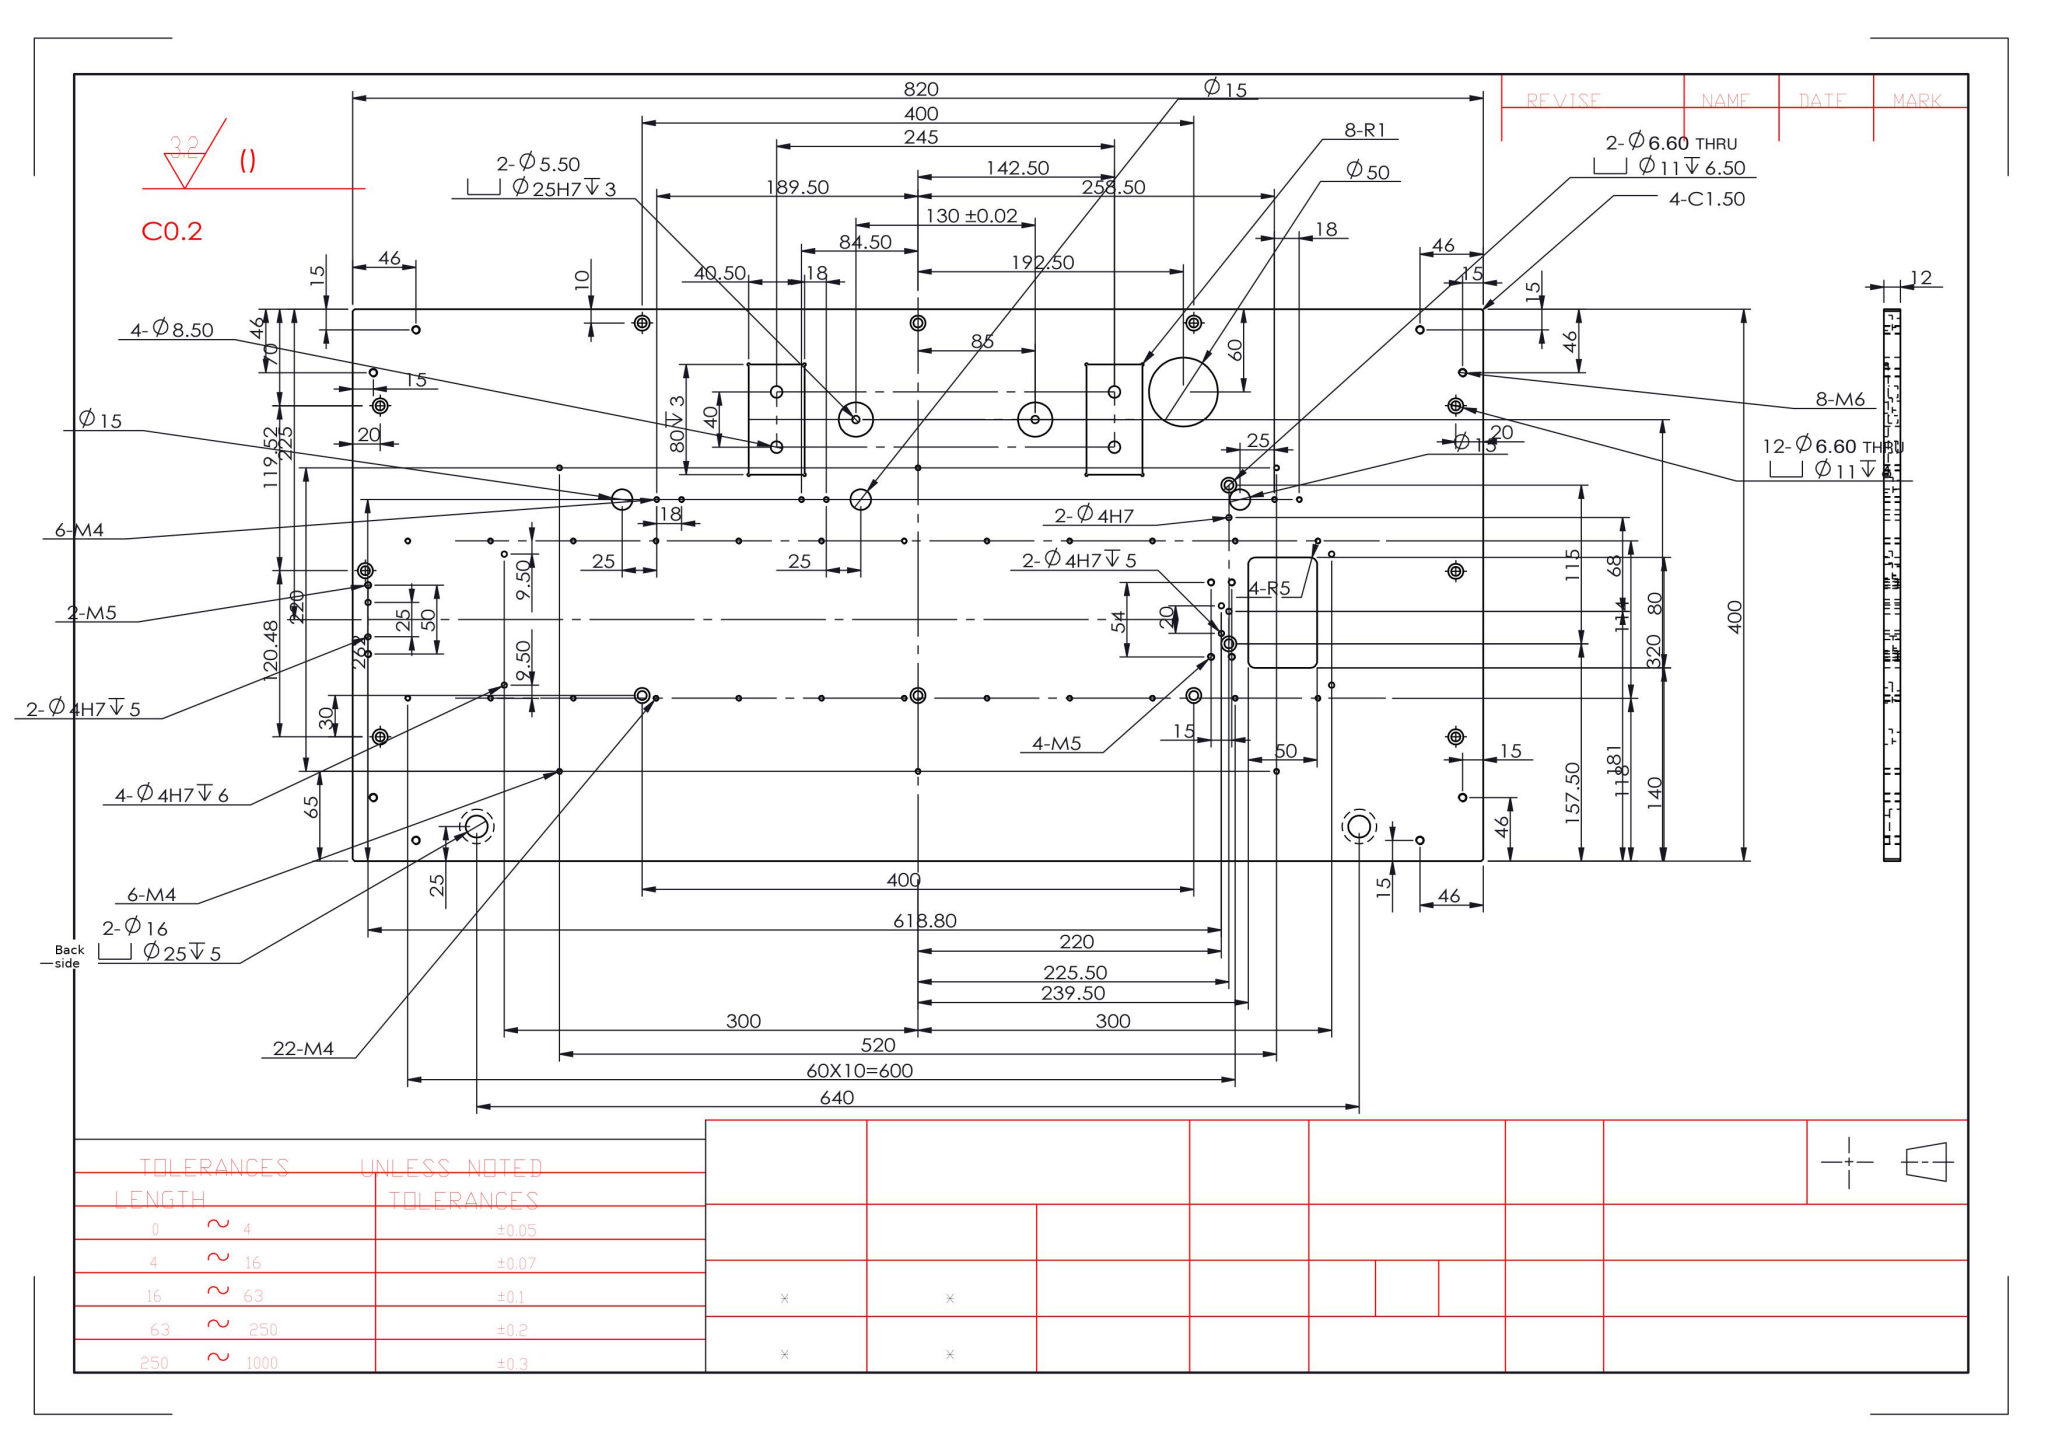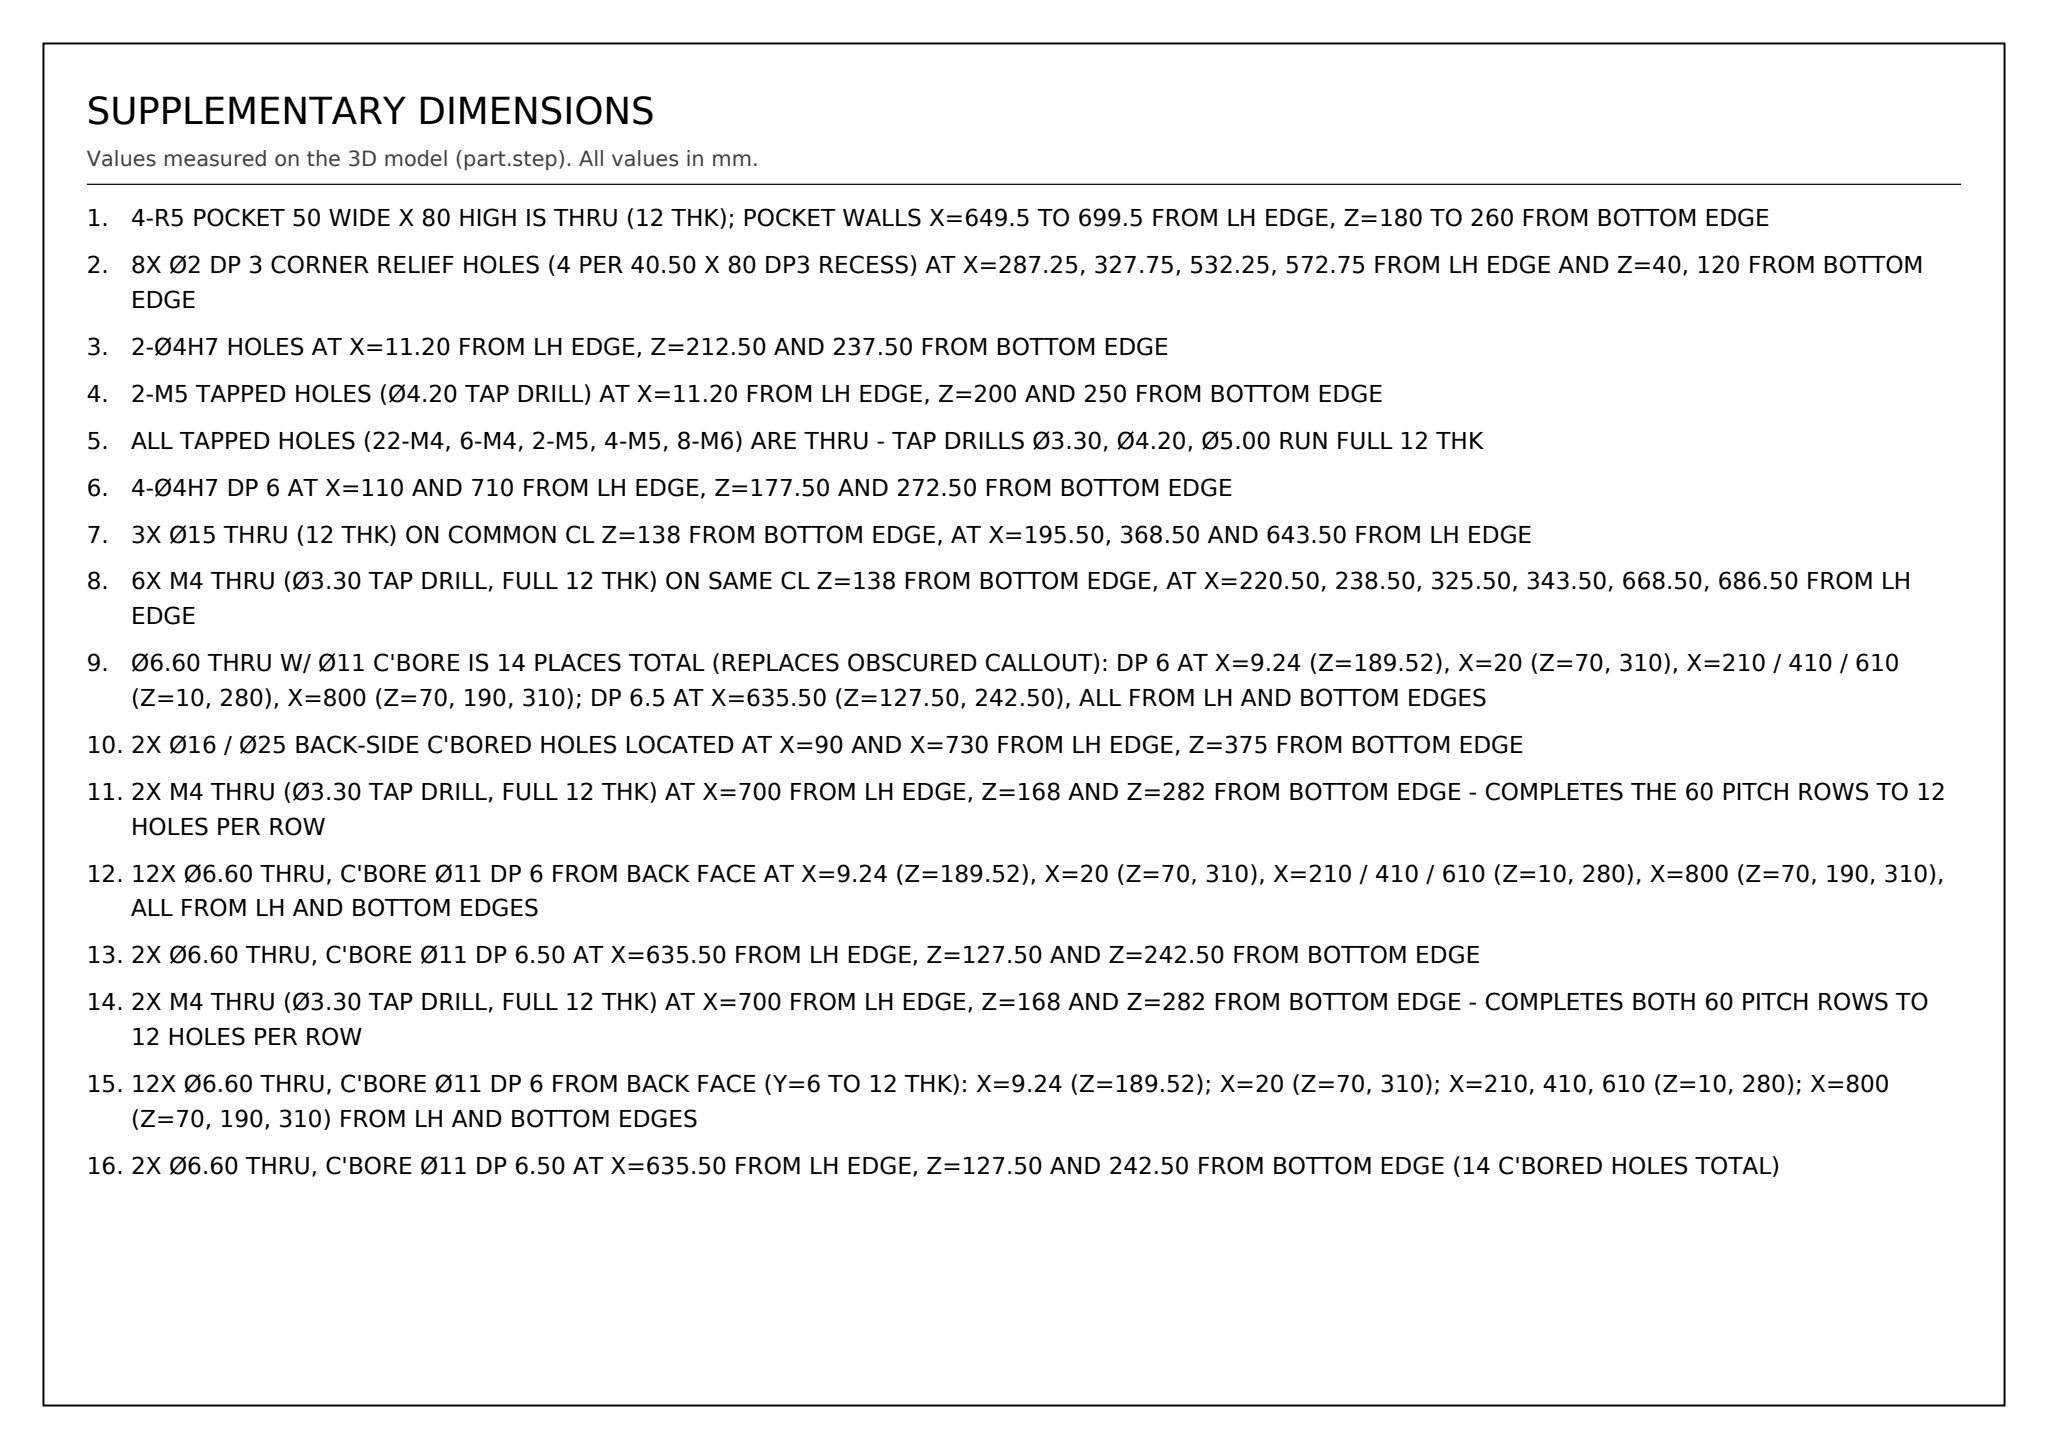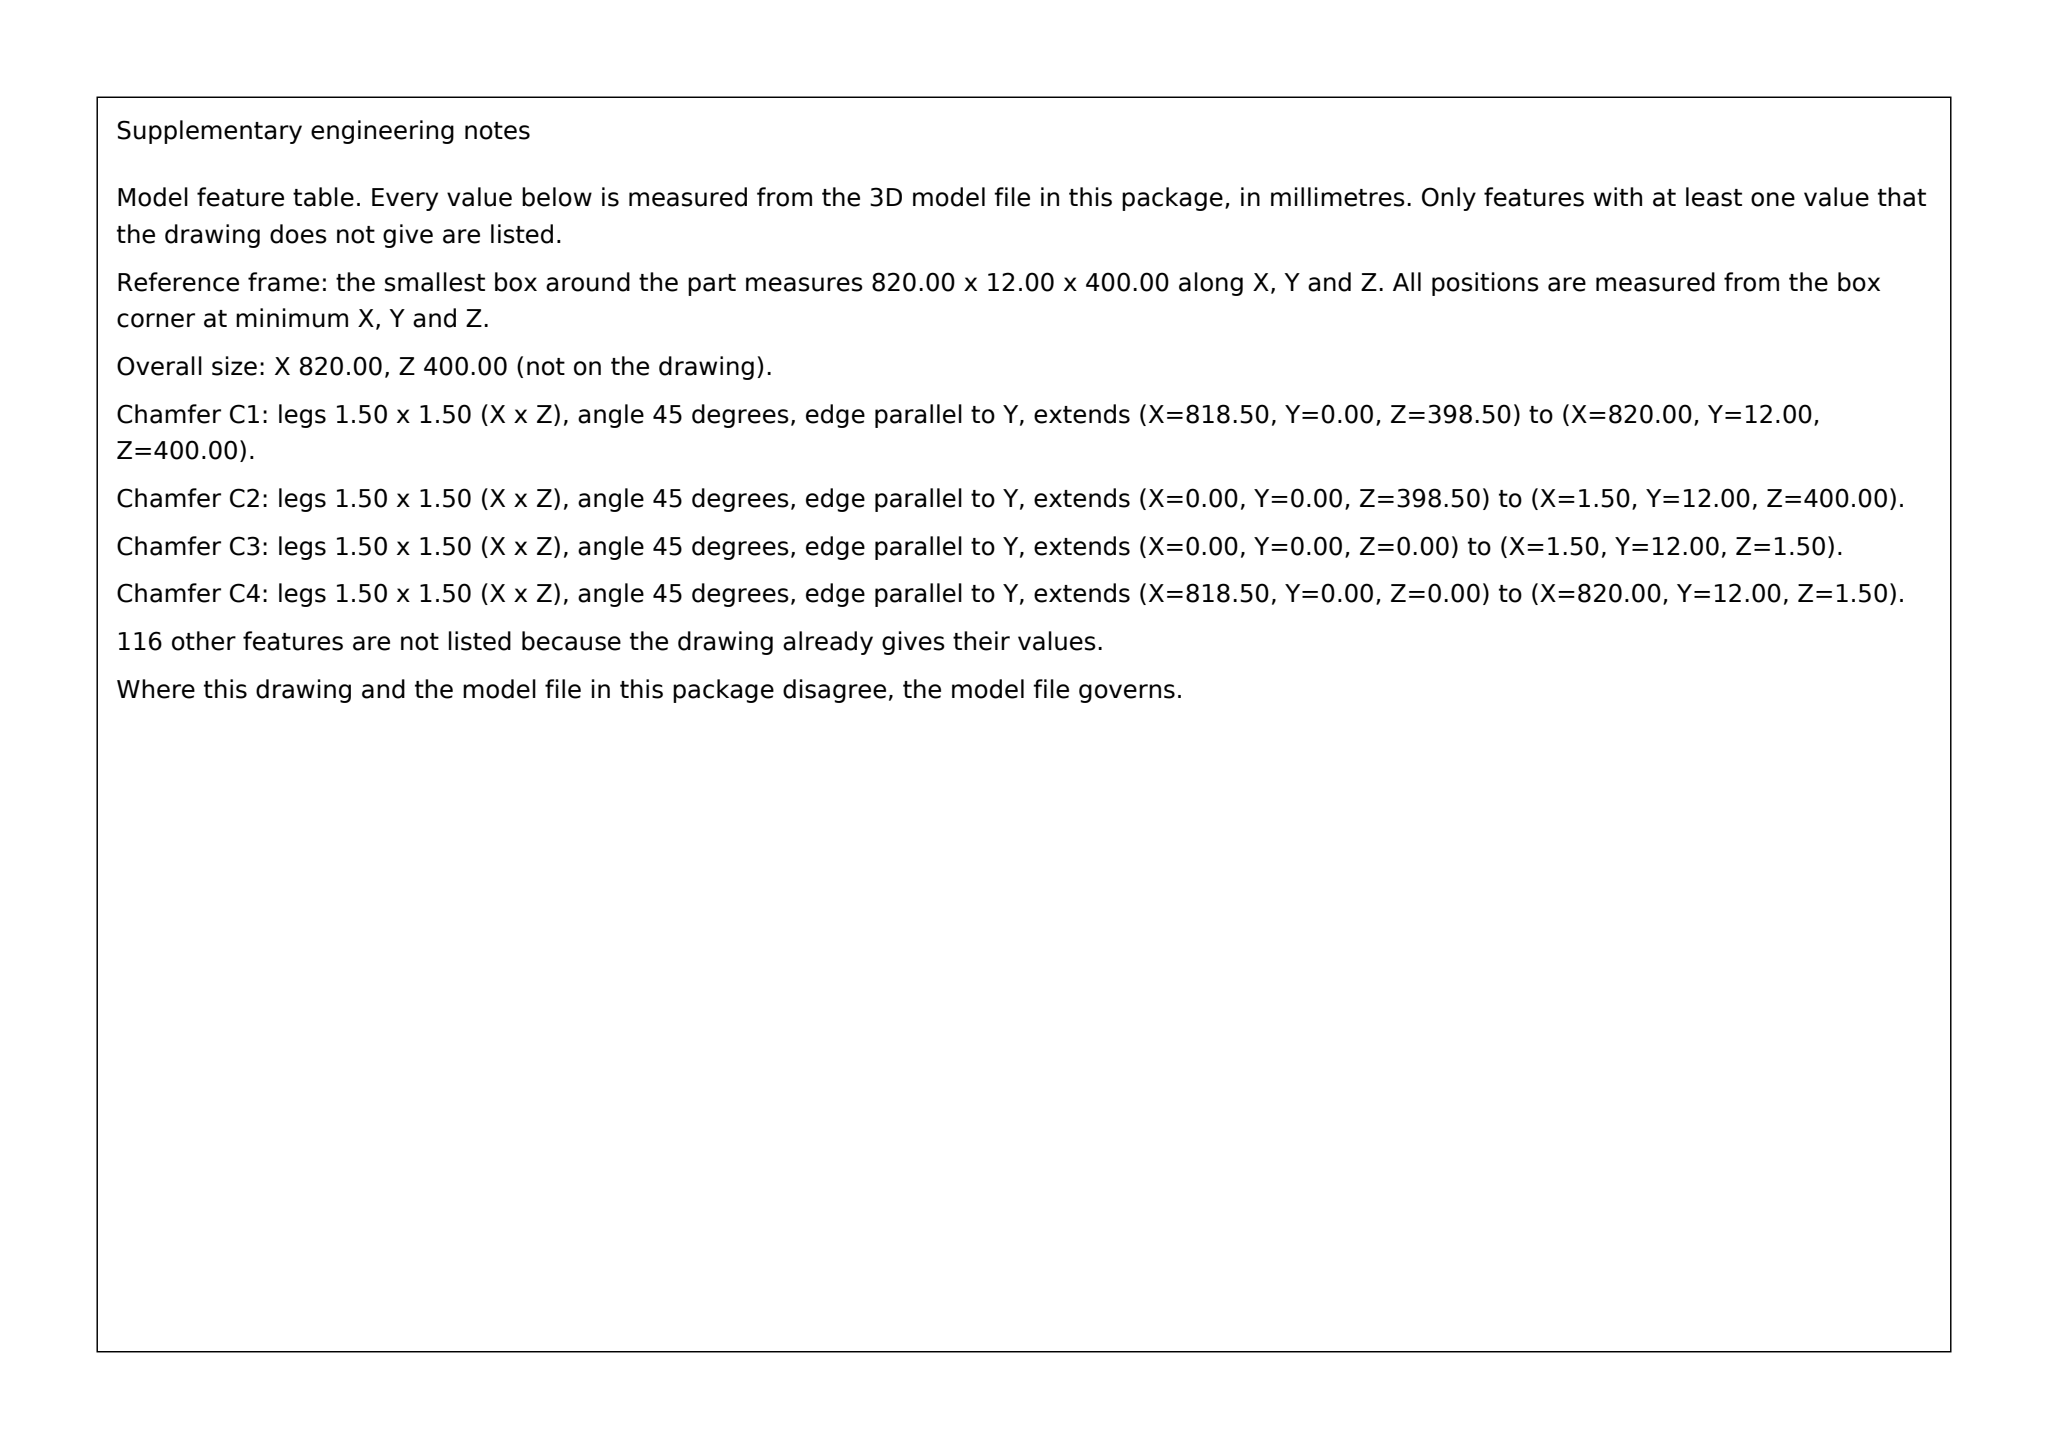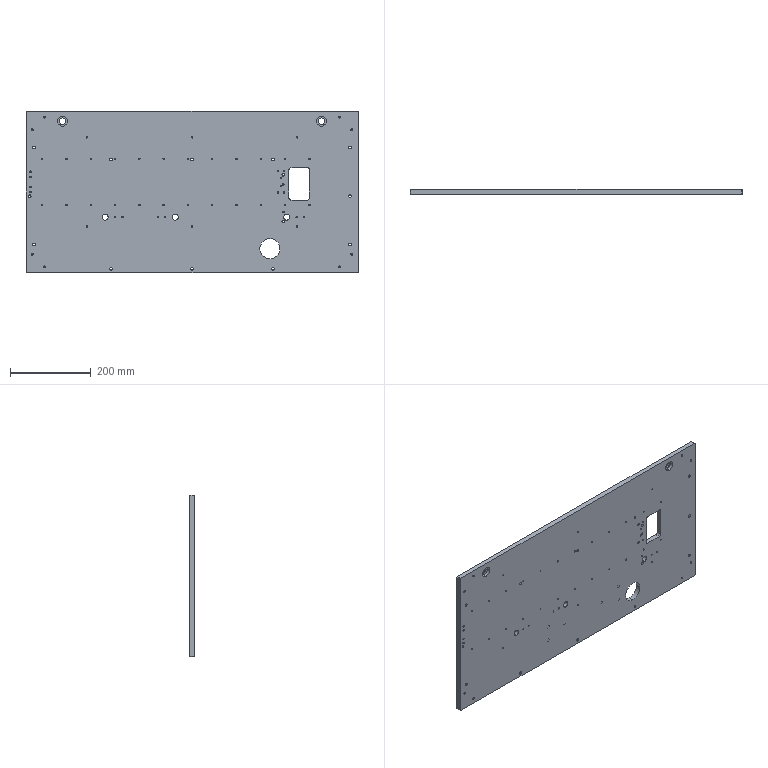Part | SolidWorks | mm | 1 solid | 276 faces | box 820 x 12 x 400 mm | volume 3805753 mm3 | cylinder 224 | plane 52 | commonest cylinder face diameters 3.3 x72 11 x28 6.6 x28 4 x20 5 x16 4.2 x12 2 x12 25 x8
Drawing notes:
4-R5 POCKET 50 WIDE X 80 HIGH IS THRU (12 THK); POCKET WALLS X=649.5 TO 699.5 FROM LH EDGE, Z=180 TO 260 FROM BOTTOM EDGE | from the solid: axis_planes x=649.5 & x=699.5, z=180 & z=260 (count 1 each); bbox_xyz y=12 with no intermediate y floor plane for the pocket
8X Ø2 DP 3 CORNER RELIEF HOLES (4 PER 40.50 X 80 DP3 RECESS) AT X=287.25, 327.75, 532.25, 572.75 FROM LH EDGE AND Z=40, 120 FROM BOTTOM EDGE | from the solid: cylinders dia 2.0, axis y, length 3.0 at (287.25/327.75/532.25/572.75, z=40 and z=120)
2-Ø4H7 HOLES AT X=11.20 FROM LH EDGE, Z=212.50 AND 237.50 FROM BOTTOM EDGE | from the solid: cylinders dia 4.0 axis y at (11.2,212.5) and (11.2,237.5)
2-M5 TAPPED HOLES (Ø4.20 TAP DRILL) AT X=11.20 FROM LH EDGE, Z=200 AND 250 FROM BOTTOM EDGE | from the solid: cylinders dia 4.2 axis y at (11.2,200) and (11.2,250), length 12
ALL TAPPED HOLES (22-M4, 6-M4, 2-M5, 4-M5, 8-M6) ARE THRU - TAP DRILLS Ø3.30, Ø4.20, Ø5.00 RUN FULL 12 THK | from the solid: cylinders dia 3.3, 4.2 and 5.0 axis y all have length 12.0 (plate thickness bbox y = 12.0)
4-Ø4H7 DP 6 AT X=110 AND 710 FROM LH EDGE, Z=177.50 AND 272.50 FROM BOTTOM EDGE | from the solid: cylinders dia 4.0 axis y at (110,177.5),(110,272.5),(710,177.5),(710,272.5), length 6.0
3X Ø15 THRU (12 THK) ON COMMON CL Z=138 FROM BOTTOM EDGE, AT X=195.50, 368.50 AND 643.50 FROM LH EDGE | from the solid: hole/bore dia 15, axis y, at [195.5,-,138], [368.5,-,138], [643.5,-,138], from 0 to 12
6X M4 THRU (Ø3.30 TAP DRILL, FULL 12 THK) ON SAME CL Z=138 FROM BOTTOM EDGE, AT X=220.50, 238.50, 325.50, 343.50, 668.50, 686.50 FROM LH EDGE | from the solid: hole/bore dia 3.3, axis y, at z=138 for x=220.5, 238.5, 325.5, 343.5, 668.5, 686.5, from 0 to 12
Ø6.60 THRU W/ Ø11 C'BORE IS 14 PLACES TOTAL (REPLACES OBSCURED CALLOUT): DP 6 AT X=9.24 (Z=189.52), X=20 (Z=70, 310), X=210 / 410 / 610 (Z=10, 280), X=800 (Z=70, 190, 310); DP 6.5 AT X=635.50 (Z=127.50, 242.50), ALL FROM LH AND BOTTOM EDGES | from the solid: all hole/bore dia 11 entries, axis y (14 instances), from 6 to 12 except the two at x=635.5 from 5.5 to 12
2X Ø16 / Ø25 BACK-SIDE C'BORED HOLES LOCATED AT X=90 AND X=730 FROM LH EDGE, Z=375 FROM BOTTOM EDGE | from the solid: hole/bore dia 16 and dia 25, axis y, axis positions [90,-,375] and [730,-,375]
2X M4 THRU (Ø3.30 TAP DRILL, FULL 12 THK) AT X=700 FROM LH EDGE, Z=168 AND Z=282 FROM BOTTOM EDGE - COMPLETES THE 60 PITCH ROWS TO 12 HOLES PER ROW | from the solid: cylinders: hole/bore Ø3.3, axis y, at [700, -, 168] and [700, -, 282], from y=0 to y=12 (THRU)
12X Ø6.60 THRU, C'BORE Ø11 DP 6 FROM BACK FACE AT X=9.24 (Z=189.52), X=20 (Z=70, 310), X=210 / 410 / 610 (Z=10, 280), X=800 (Z=70, 190, 310), ALL FROM LH AND BOTTOM EDGES | from the solid: cylinders: hole/bore Ø11, axis y, from y=6.0 to y=12.0 at [9.2,189.5], [20,70], [20,310], [210,10], [210,280], [410,10], [410,280], [610,10], [610,280], [800,70], [800,190], [800,310]
2X Ø6.60 THRU, C'BORE Ø11 DP 6.50 AT X=635.50 FROM LH EDGE, Z=127.50 AND Z=242.50 FROM BOTTOM EDGE | from the solid: cylinders: hole/bore Ø11, axis y, from y=5.5 to y=12.0 at [635.5,-,127.5] and [635.5,-,242.5]
2X M4 THRU (Ø3.30 TAP DRILL, FULL 12 THK) AT X=700 FROM LH EDGE, Z=168 AND Z=282 FROM BOTTOM EDGE - COMPLETES BOTH 60 PITCH ROWS TO 12 HOLES PER ROW | from the solid: cylinders: Ø3.3 axis y at [700,null,168] and [700,null,282], from y=0 to y=12 (thru)
12X Ø6.60 THRU, C'BORE Ø11 DP 6 FROM BACK FACE (Y=6 TO 12 THK): X=9.24 (Z=189.52); X=20 (Z=70, 310); X=210, 410, 610 (Z=10, 280); X=800 (Z=70, 190, 310) FROM LH AND BOTTOM EDGES | from the solid: twelve 'hole/bore' Ø11.0 cylinders, axis y, from 6.0 to 12.0 at those x/z positions
2X Ø6.60 THRU, C'BORE Ø11 DP 6.50 AT X=635.50 FROM LH EDGE, Z=127.50 AND 242.50 FROM BOTTOM EDGE (14 C'BORED HOLES TOTAL) | from the solid: 'hole/bore' Ø11.0 axis y at [635.5,-,127.5] and [635.5,-,242.5], from 5.5 to 12.0 (6.5 deep); 14 Ø11 bores total in model
build123d program:
from build123d import *

# Parameters (mm, degrees)
SKETCH1_2_W                                          = 820
SKETCH1_2_H                                          = 400
EXTRUDE1_DEPTH                                       = 12
CHAMFER1_SIZE                                        = 1.5
CYLINDRICAL_COUNTERSUNK_HOLE_FOR_M6_SOCK_D           = 6.6
CYLINDRICAL_COUNTERSUNK_HOLE_FOR_M6_SOCK_CBORE_D     = 11
CYLINDRICAL_COUNTERSUNK_HOLE_FOR_M6_SOCK_CBORE_DEPTH = 6
SKETCH5_R                                            = 2.75
SKETCH5_R_2                                          = 4.25
EXTRUDE4_DEPTH                                       = 10
SKETCH6_R                                            = 12.5
SKETCH6_W                                            = 40.5
SKETCH6_H                                            = 80
EXTRUDE5_DEPTH                                       = 3
SKETCH7_R                                            = 25
EXTRUDE6_DEPTH                                       = 15
M6_TAPPED_HOLE1_D                                    = 5
SKETCH14_R                                           = 1
EXTRUDE8_DEPTH                                       = 3
SKETCH15_R                                           = 8
EXTRUDE9_DEPTH                                       = 457.338
SKETCH16_R                                           = 12.5
EXTRUDE10_DEPTH                                      = 8
M4_TAPPED_HOLE1_D                                    = 3.3
LPATTERN1_COUNT                                      = 12
LPATTERN1_PITCH                                      = 60
M4_TAPPED_HOLE3_D                                    = 3.3
SKETCH36_R                                           = 2
SKETCH36_W                                           = 50
SKETCH36_H                                           = 80
CUT_EXTRUDE1_DEPTH                                   = 457.338
SKETCH37_R                                           = 2
CUT_EXTRUDE2_DEPTH                                   = 457.338
M5_TAPPED_HOLE1_D                                    = 4.2
M6_HEX_SOCKET_HEAD_CAP_SCREW_CBORE1_D                = 6.6
M6_HEX_SOCKET_HEAD_CAP_SCREW_CBORE1_CBORE_D          = 11
M6_HEX_SOCKET_HEAD_CAP_SCREW_CBORE1_CBORE_DEPTH      = 6.5
M4_TAPPED_HOLE2_D                                    = 3.3
FILLET1_R                                            = 5
SKETCH42_R                                           = 7.5
CUT_EXTRUDE3_DEPTH                                   = 457.338
SKETCH43_R                                           = 2
CUT_EXTRUDE4_DEPTH                                   = 6


with BuildPart() as part:
    # Sketch1_2 → Extrude1 (new body)
    with BuildSketch(Plane(origin=(0, 0, 0), x_dir=(1, 0, 0), z_dir=(0, 1, 0))):
        Rectangle(SKETCH1_2_W, SKETCH1_2_H)
    extrude(amount=EXTRUDE1_DEPTH)

    # Chamfer1
    chamfer1_edges = [part.edges().sort_by_distance(p)[0] for p in [
        (-410, 6, -200),
        (410, 6, -200),
        (410, 6, 200),
        (-410, 6, 200),
    ]]
    chamfer(chamfer1_edges, length=CHAMFER1_SIZE)

    # Cylindrical Countersunk Hole for M6 Sock (through all)
    with Locations(Plane(origin=(0, 12, 0), x_dir=(-1, 0, 0), z_dir=(0, 1, 0))):
        with Locations((200, -190), (0, -190), (-200, -190), (-390, -130), (-390, -10), (-390, 110), (390, 110), (400.763, -10.484), (390, -130), (200, 80), (0, 80), (-200, 80)):
            CounterBoreHole(CYLINDRICAL_COUNTERSUNK_HOLE_FOR_M6_SOCK_D / 2, CYLINDRICAL_COUNTERSUNK_HOLE_FOR_M6_SOCK_CBORE_D / 2, CYLINDRICAL_COUNTERSUNK_HOLE_FOR_M6_SOCK_CBORE_DEPTH)

    # Sketch5 → Extrude4 (cut)
    with BuildSketch(Plane(origin=(0, 12, 0), x_dir=(-1, 0, 0), z_dir=(0, 1, 0))):
        with Locations(Location((45, -120, 0), (0, 0, 90))):
            Circle(SKETCH5_R)
        with Locations(Location((-85, -120, 0), (0, 0, 90))):
            Circle(SKETCH5_R)
        with Locations(Location((102.5, -140, 0), (0, 0, 90))):
            Circle(SKETCH5_R_2)
        with Locations(Location((102.5, -100, 0), (0, 0, 90))):
            Circle(SKETCH5_R_2)
        with Locations(Location((-142.5, -100, 0), (0, 0, 90))):
            Circle(SKETCH5_R_2)
        with Locations(Location((-142.5, -140, 0), (0, 0, 90))):
            Circle(SKETCH5_R_2)
    extrude(amount=-EXTRUDE4_DEPTH, mode=Mode.SUBTRACT)

    # Sketch6 → Extrude5 (cut)
    with BuildSketch(Plane(origin=(0, 12, 0), x_dir=(-1, 0, 0), z_dir=(0, 1, 0))):
        with Locations(Location((45, -120, 0), (0, 0, 90))):
            Circle(SKETCH6_R)
        with Locations(Location((-85, -120, 0), (0, 0, 90))):
            Circle(SKETCH6_R)
        with Locations((102.5, -120)):
            Rectangle(SKETCH6_W, SKETCH6_H)
        with Locations((-142.5, -120)):
            Rectangle(SKETCH6_W, SKETCH6_H)
    extrude(amount=-EXTRUDE5_DEPTH, mode=Mode.SUBTRACT)

    # Sketch7 → Extrude6 (cut)
    with BuildSketch(Plane(origin=(0, 12, 0), x_dir=(-1, 0, 0), z_dir=(0, 1, 0))):
        with Locations(Location((-192.5, -140, 0), (0, 0, 90))):
            Circle(SKETCH7_R)
    extrude(amount=-EXTRUDE6_DEPTH, mode=Mode.SUBTRACT)

    # M6 Tapped Hole1 (through all)
    with Locations(Plane(origin=(-395, 12, -154), x_dir=(0, 0, 1), z_dir=(0, 1, 0))):
        with Locations((0, 0), (-31, 31), (-31, 759), (0, 790), (308, 790), (308, 0), (339, 31), (339, 759)):
            Hole(M6_TAPPED_HOLE1_D / 2)

    # Sketch14 → Extrude8 (cut)
    with BuildSketch(Plane(origin=(0, 12, 0), x_dir=(-1, 0, 0), z_dir=(0, 1, 0))):
        with Locations((82.25, -160)):
            Circle(SKETCH14_R)
        with Locations((122.75, -160)):
            Circle(SKETCH14_R)
        with Locations((82.25, -80)):
            Circle(SKETCH14_R)
        with Locations((122.75, -80)):
            Circle(SKETCH14_R)
        with Locations((-122.25, -160)):
            Circle(SKETCH14_R)
        with Locations((-162.75, -160)):
            Circle(SKETCH14_R)
        with Locations((-122.25, -80)):
            Circle(SKETCH14_R)
        with Locations((-162.75, -80)):
            Circle(SKETCH14_R)
    extrude(amount=-EXTRUDE8_DEPTH, mode=Mode.SUBTRACT)

    # Sketch15 → Extrude9 (cut, through all)
    with BuildSketch(Plane(origin=(0, 12, 0), x_dir=(-1, 0, 0), z_dir=(0, 1, 0))):
        with Locations(Location((-320, 175, 0), (0, 0, 90))):
            Circle(SKETCH15_R)
        with Locations(Location((320, 175, 0), (0, 0, 90))):
            Circle(SKETCH15_R)
    extrude(amount=-EXTRUDE9_DEPTH, mode=Mode.SUBTRACT)

    # Sketch16 → Extrude10 (cut)
    with BuildSketch(Plane.XZ):
        with Locations(Location((320, 175, 0), (0, 0, 270))):
            Circle(SKETCH16_R)
        with Locations(Location((-320, 175, 0), (0, 0, 270))):
            Circle(SKETCH16_R)
    extrude(amount=-EXTRUDE10_DEPTH, mode=Mode.SUBTRACT)

    # M4 Tapped Hole1 (through all)
    with Locations(Plane(origin=(-370, 12, 82), x_dir=(0, 0, 1), z_dir=(0, 1, 0))):
        with Locations((0, 0), (-114, 0)):
            m4_tapped_hole1 = Hole(M4_TAPPED_HOLE1_D / 2)

    # LPattern1: M4 Tapped Hole1 ×12
    with Locations(*[(i * LPATTERN1_PITCH, 0, 0) for i in range(1, LPATTERN1_COUNT)]):
        add(m4_tapped_hole1, mode=Mode.SUBTRACT)

    # M4 Tapped Hole3 (through all)
    with Locations(Plane(origin=(-189.5, 12, -62), x_dir=(0, 0, 1), z_dir=(0, 1, 0))):
        with Locations((0, 0), (0, 18), (0, 105), (0, 123), (0, 448), (0, 466)):
            Hole(M4_TAPPED_HOLE3_D / 2)

    # Sketch36 → Cut-Extrude1 (cut, through all)
    with BuildSketch(Plane(origin=(0, 12, 0), x_dir=(1, 0, 0), z_dir=(0, 1, 0))):
        with Locations(Location((225.5, 49, 0), (0, 0, 270))):
            Circle(SKETCH36_R)
        with Locations(Location((225.5, -19, 0), (0, 0, 270))):
            Circle(SKETCH36_R)
        with Locations((264.5, -20)):
            Rectangle(SKETCH36_W, SKETCH36_H)
    extrude(amount=-CUT_EXTRUDE1_DEPTH, mode=Mode.SUBTRACT)

    # Sketch37 → Cut-Extrude2 (cut, through all)
    with BuildSketch(Plane(origin=(0, 12, 0), x_dir=(-1, 0, 0), z_dir=(0, 1, 0))):
        with Locations(Location((-220, 15, 0), (0, 0, 90))):
            Circle(SKETCH37_R)
        with Locations(Location((-220, 35, 0), (0, 0, 90))):
            Circle(SKETCH37_R)
        with Locations(Location((398.8, 12.5, 0), (0, 0, 90))):
            Circle(SKETCH37_R)
        with Locations(Location((398.8, 37.5, 0), (0, 0, 90))):
            Circle(SKETCH37_R)
    extrude(amount=-CUT_EXTRUDE2_DEPTH, mode=Mode.SUBTRACT)

    # M5 Tapped Hole1 (through all)
    with Locations(Plane(origin=(-398.8, 12, 0), x_dir=(0, 0, 1), z_dir=(0, 1, 0))):
        with Locations((0, 0), (50, 0), (-2, 611.3), (-2, 626.3), (52, 611.3), (52, 626.3)):
            Hole(M5_TAPPED_HOLE1_D / 2)

    # M6 Hex Socket Head Cap Screw CBORE1 (through all)
    with Locations(Plane(origin=(225.5, 12, -72.5), x_dir=(0, 0, 1), z_dir=(0, 1, 0))):
        with Locations((0, 0), (115, 0)):
            CounterBoreHole(M6_HEX_SOCKET_HEAD_CAP_SCREW_CBORE1_D / 2, M6_HEX_SOCKET_HEAD_CAP_SCREW_CBORE1_CBORE_D / 2, M6_HEX_SOCKET_HEAD_CAP_SCREW_CBORE1_CBORE_DEPTH)

    # M4 Tapped Hole2 (through all)
    with Locations(Plane(origin=(-260, 12, 135), x_dir=(0, 0, 1), z_dir=(0, 1, 0))):
        with Locations((0, 0), (0, 260), (0, 520), (-220, 520), (-220, 260), (-220, 0)):
            Hole(M4_TAPPED_HOLE2_D / 2)

    # Fillet1
    fillet1_edges = [part.edges().sort_by_distance(p)[0] for p in [
        (239.5, 6, 60),
        (239.5, 6, -20),
        (289.5, 6, -20),
        (289.5, 6, 60),
    ]]
    fillet(fillet1_edges, radius=FILLET1_R)

    # Sketch42 → Cut-Extrude3 (cut, through all)
    with BuildSketch(Plane(origin=(0, 12, 0), x_dir=(1, 0, 0), z_dir=(0, 1, 0))):
        with Locations(Location((233.5, 62, 0), (0, 0, 270))):
            Circle(SKETCH42_R)
        with Locations(Location((-41.5, 62, 0), (0, 0, 270))):
            Circle(SKETCH42_R)
        with Locations(Location((-214.5, 62, 0), (0, 0, 270))):
            Circle(SKETCH42_R)
    extrude(amount=-CUT_EXTRUDE3_DEPTH, mode=Mode.SUBTRACT)

    # Sketch43 → Cut-Extrude4 (cut)
    with BuildSketch(Plane(origin=(0, 12, 0), x_dir=(1, 0, 0), z_dir=(0, 1, 0))):
        with Locations(Location((300, 22.5, 0), (0, 0, 270))):
            Circle(SKETCH43_R)
        with Locations(Location((-300, 22.5, 0), (0, 0, 270))):
            Circle(SKETCH43_R)
        with Locations(Location((-300, -72.5, 0), (0, 0, 270))):
            Circle(SKETCH43_R)
        with Locations(Location((300, -72.5, 0), (0, 0, 270))):
            Circle(SKETCH43_R)
    extrude(amount=-CUT_EXTRUDE4_DEPTH, mode=Mode.SUBTRACT)


solid = part.part